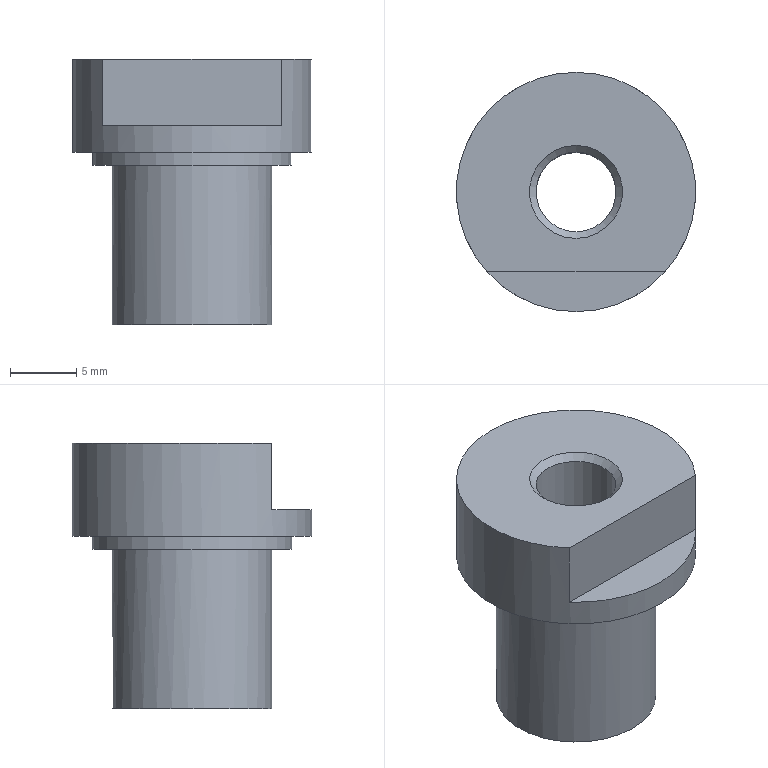Component | NX | REPL_DRILL_BUSH | 1 solid | 12 faces | box 18 x 18 x 20 mm | volume 2605 mm3 | plane 6 | cylinder 4 | cone 2 | commonest cylinder face diameters 12 x1 15 x1 18 x1 6 x1
STEP:
#1=CARTESIAN_POINT('',(0.,0.,0.));
#2=DIRECTION('',(0.,0.,1.));
#3=DIRECTION('',(1.,0.,0.));
#4=AXIS2_PLACEMENT_3D('',#1,#2,#3);
#5=CARTESIAN_POINT('',(11.228,-14.027,-173.719));
#6=VERTEX_POINT('',#5);
#7=CARTESIAN_POINT('',(11.228,-17.527,-173.719));
#8=DIRECTION('',(0.,0.,1.));
#9=DIRECTION('',(0.,1.,0.));
#10=AXIS2_PLACEMENT_3D('',#7,#8,#9);
#11=CIRCLE('',#10,3.5);
#12=CARTESIAN_POINT('',(11.228,-17.527,-173.719));
#13=DIRECTION('',(0.,0.,-1.));
#14=DIRECTION('',(0.,1.,0.));
#15=AXIS2_PLACEMENT_3D('',#12,#13,#14);
#16=PLANE('',#15);
#17=CARTESIAN_POINT('',(3.5,0.));
#18=CARTESIAN_POINT('',(3.5,-6.062));
#19=CARTESIAN_POINT('',(-1.75,-3.031));
#20=CARTESIAN_POINT('',(-7.,-0.));
#21=CARTESIAN_POINT('',(-1.75,3.031));
#22=CARTESIAN_POINT('',(3.5,6.062));
#23=CARTESIAN_POINT('',(3.5,0.));
#24=(BOUNDED_CURVE()B_SPLINE_CURVE(2,(#17,#18,#19,#20,#21,#22,#23),.UNSPECIFIED.,.T.,.F.)B_SPLINE_CURVE_WITH_KNOTS((1,2,2,2,2,1),(-2.094,0.,2.094,4.189,6.283,8.378),.UNSPECIFIED.)CURVE()GEOMETRIC_REPRESENTATION_ITEM()RATIONAL_B_SPLINE_CURVE((1.,0.5,1.,0.5,1.,0.5,1.))REPRESENTATION_ITEM(''));
#25=(GEOMETRIC_REPRESENTATION_CONTEXT(2)PARAMETRIC_REPRESENTATION_CONTEXT()REPRESENTATION_CONTEXT('',''));
#26=DEFINITIONAL_REPRESENTATION('',(#24),#25);
#27=PCURVE('',#16,#26);
#28=CARTESIAN_POINT('',(11.228,-17.527,-173.219));
#29=DIRECTION('',(0.,0.,-1.));
#30=DIRECTION('',(0.,1.,0.));
#31=AXIS2_PLACEMENT_3D('',#28,#29,#30);
#32=CONICAL_SURFACE('',#31,3.,0.7854);
#33=CARTESIAN_POINT('',(6.283,0.5));
#34=DIRECTION('',(-1.,0.));
#35=VECTOR('',#34,1.);
#36=LINE('',#33,#35);
#37=(GEOMETRIC_REPRESENTATION_CONTEXT(2)PARAMETRIC_REPRESENTATION_CONTEXT()REPRESENTATION_CONTEXT('',''));
#38=DEFINITIONAL_REPRESENTATION('',(#36),#37);
#39=PCURVE('',#32,#38);
#40=SURFACE_CURVE('',#11,(#27,#39),.PCURVE_S1.);
#41=EDGE_CURVE('',#6,#6,#40,.T.);
#42=ORIENTED_EDGE('',*,*,#41,.T.);
#43=EDGE_LOOP('',(#42));
#44=FACE_BOUND('',#43,.T.);
#45=CARTESIAN_POINT('',(11.228,-23.527,-173.719));
#46=VERTEX_POINT('',#45);
#47=CARTESIAN_POINT('',(11.228,-17.527,-173.719));
#48=DIRECTION('',(0.,0.,1.));
#49=DIRECTION('',(0.,-1.,0.));
#50=AXIS2_PLACEMENT_3D('',#47,#48,#49);
#51=CIRCLE('',#50,6.);
#52=CARTESIAN_POINT('',(-6.,0.));
#53=CARTESIAN_POINT('',(-6.,10.392));
#54=CARTESIAN_POINT('',(3.,5.196));
#55=CARTESIAN_POINT('',(12.,0.));
#56=CARTESIAN_POINT('',(3.,-5.196));
#57=CARTESIAN_POINT('',(-6.,-10.392));
#58=CARTESIAN_POINT('',(-6.,0.));
#59=(BOUNDED_CURVE()B_SPLINE_CURVE(2,(#52,#53,#54,#55,#56,#57,#58),.UNSPECIFIED.,.T.,.F.)B_SPLINE_CURVE_WITH_KNOTS((1,2,2,2,2,1),(-2.094,0.,2.094,4.189,6.283,8.378),.UNSPECIFIED.)CURVE()GEOMETRIC_REPRESENTATION_ITEM()RATIONAL_B_SPLINE_CURVE((1.,0.5,1.,0.5,1.,0.5,1.))REPRESENTATION_ITEM(''));
#60=(GEOMETRIC_REPRESENTATION_CONTEXT(2)PARAMETRIC_REPRESENTATION_CONTEXT()REPRESENTATION_CONTEXT('',''));
#61=DEFINITIONAL_REPRESENTATION('',(#59),#60);
#62=PCURVE('',#16,#61);
#63=CARTESIAN_POINT('',(11.228,-17.527,-173.719));
#64=DIRECTION('',(0.,0.,1.));
#65=DIRECTION('',(0.,-1.,0.));
#66=AXIS2_PLACEMENT_3D('',#63,#64,#65);
#67=CYLINDRICAL_SURFACE('',#66,6.);
#68=CARTESIAN_POINT('',(0.,0.));
#69=DIRECTION('',(1.,0.));
#70=VECTOR('',#69,1.);
#71=LINE('',#68,#70);
#72=(GEOMETRIC_REPRESENTATION_CONTEXT(2)PARAMETRIC_REPRESENTATION_CONTEXT()REPRESENTATION_CONTEXT('',''));
#73=DEFINITIONAL_REPRESENTATION('',(#71),#72);
#74=PCURVE('',#67,#73);
#75=SURFACE_CURVE('',#51,(#62,#74),.PCURVE_S1.);
#76=EDGE_CURVE('',#46,#46,#75,.T.);
#77=ORIENTED_EDGE('',*,*,#76,.F.);
#78=EDGE_LOOP('',(#77));
#79=FACE_BOUND('',#78,.T.);
#80=ADVANCED_FACE('',(#44,#79),#16,.T.);
#81=CARTESIAN_POINT('',(11.228,-23.527,-161.719));
#82=VERTEX_POINT('',#81);
#83=CARTESIAN_POINT('',(11.228,-11.527,-161.719));
#84=VERTEX_POINT('',#83);
#85=CARTESIAN_POINT('',(11.228,-17.527,-161.719));
#86=DIRECTION('',(0.,0.,1.));
#87=DIRECTION('',(0.,1.,0.));
#88=AXIS2_PLACEMENT_3D('',#85,#86,#87);
#89=CIRCLE('',#88,6.);
#90=CARTESIAN_POINT('',(-3.142,12.));
#91=DIRECTION('',(1.,0.));
#92=VECTOR('',#91,1.);
#93=LINE('',#90,#92);
#94=(GEOMETRIC_REPRESENTATION_CONTEXT(2)PARAMETRIC_REPRESENTATION_CONTEXT()REPRESENTATION_CONTEXT('',''));
#95=DEFINITIONAL_REPRESENTATION('',(#93),#94);
#96=PCURVE('',#67,#95);
#97=CARTESIAN_POINT('',(11.228,-17.527,-161.719));
#98=DIRECTION('',(0.,0.,-1.));
#99=DIRECTION('',(0.,1.,0.));
#100=AXIS2_PLACEMENT_3D('',#97,#98,#99);
#101=PLANE('',#100);
#102=CARTESIAN_POINT('',(6.,0.));
#103=CARTESIAN_POINT('',(6.,-10.392));
#104=CARTESIAN_POINT('',(-3.,-5.196));
#105=CARTESIAN_POINT('',(-12.,-0.));
#106=CARTESIAN_POINT('',(-3.,5.196));
#107=CARTESIAN_POINT('',(6.,10.392));
#108=CARTESIAN_POINT('',(6.,0.));
#109=(BOUNDED_CURVE()B_SPLINE_CURVE(2,(#102,#103,#104,#105,#106,#107,#108),.UNSPECIFIED.,.T.,.F.)B_SPLINE_CURVE_WITH_KNOTS((1,2,2,2,2,1),(-2.094,0.,2.094,4.189,6.283,8.378),.UNSPECIFIED.)CURVE()GEOMETRIC_REPRESENTATION_ITEM()RATIONAL_B_SPLINE_CURVE((1.,0.5,1.,0.5,1.,0.5,1.))REPRESENTATION_ITEM(''));
#110=(GEOMETRIC_REPRESENTATION_CONTEXT(2)PARAMETRIC_REPRESENTATION_CONTEXT()REPRESENTATION_CONTEXT('',''));
#111=DEFINITIONAL_REPRESENTATION('',(#109),#110);
#112=PCURVE('',#101,#111);
#113=SURFACE_CURVE('',#89,(#96,#112),.PCURVE_S1.);
#114=EDGE_CURVE('',#82,#84,#113,.T.);
#115=ORIENTED_EDGE('',*,*,#114,.F.);
#116=CARTESIAN_POINT('',(11.228,-23.527,-173.719));
#117=CARTESIAN_POINT('',(11.228,-23.527,-161.719));
#118=B_SPLINE_CURVE_WITH_KNOTS('',1,(#116,#117),.UNSPECIFIED.,.F.,.F.,(2,2),(0.,12.),.PIECEWISE_BEZIER_KNOTS.);
#119=CARTESIAN_POINT('',(0.,0.));
#120=DIRECTION('',(0.,1.));
#121=VECTOR('',#120,1.);
#122=LINE('',#119,#121);
#123=(GEOMETRIC_REPRESENTATION_CONTEXT(2)PARAMETRIC_REPRESENTATION_CONTEXT()REPRESENTATION_CONTEXT('',''));
#124=DEFINITIONAL_REPRESENTATION('',(#122),#123);
#125=PCURVE('',#67,#124);
#126=CARTESIAN_POINT('',(6.283,0.));
#127=DIRECTION('',(0.,1.));
#128=VECTOR('',#127,1.);
#129=LINE('',#126,#128);
#130=(GEOMETRIC_REPRESENTATION_CONTEXT(2)PARAMETRIC_REPRESENTATION_CONTEXT()REPRESENTATION_CONTEXT('',''));
#131=DEFINITIONAL_REPRESENTATION('',(#129),#130);
#132=PCURVE('',#67,#131);
#133=SEAM_CURVE('',#118,(#125,#132),.PCURVE_S1.);
#134=EDGE_CURVE('',#46,#82,#133,.T.);
#135=ORIENTED_EDGE('',*,*,#134,.F.);
#136=ORIENTED_EDGE('',*,*,#76,.T.);
#137=ORIENTED_EDGE('',*,*,#134,.T.);
#138=CARTESIAN_POINT('',(11.228,-17.527,-161.719));
#139=DIRECTION('',(0.,0.,1.));
#140=DIRECTION('',(0.,1.,0.));
#141=AXIS2_PLACEMENT_3D('',#138,#139,#140);
#142=CIRCLE('',#141,6.);
#143=CARTESIAN_POINT('',(3.142,12.));
#144=DIRECTION('',(1.,0.));
#145=VECTOR('',#144,1.);
#146=LINE('',#143,#145);
#147=(GEOMETRIC_REPRESENTATION_CONTEXT(2)PARAMETRIC_REPRESENTATION_CONTEXT()REPRESENTATION_CONTEXT('',''));
#148=DEFINITIONAL_REPRESENTATION('',(#146),#147);
#149=PCURVE('',#67,#148);
#150=CARTESIAN_POINT('',(6.,0.));
#151=CARTESIAN_POINT('',(6.,-10.392));
#152=CARTESIAN_POINT('',(-3.,-5.196));
#153=CARTESIAN_POINT('',(-12.,-0.));
#154=CARTESIAN_POINT('',(-3.,5.196));
#155=CARTESIAN_POINT('',(6.,10.392));
#156=CARTESIAN_POINT('',(6.,0.));
#157=(BOUNDED_CURVE()B_SPLINE_CURVE(2,(#150,#151,#152,#153,#154,#155,#156),.UNSPECIFIED.,.T.,.F.)B_SPLINE_CURVE_WITH_KNOTS((1,2,2,2,2,1),(-2.094,0.,2.094,4.189,6.283,8.378),.UNSPECIFIED.)CURVE()GEOMETRIC_REPRESENTATION_ITEM()RATIONAL_B_SPLINE_CURVE((1.,0.5,1.,0.5,1.,0.5,1.))REPRESENTATION_ITEM(''));
#158=(GEOMETRIC_REPRESENTATION_CONTEXT(2)PARAMETRIC_REPRESENTATION_CONTEXT()REPRESENTATION_CONTEXT('',''));
#159=DEFINITIONAL_REPRESENTATION('',(#157),#158);
#160=PCURVE('',#101,#159);
#161=SURFACE_CURVE('',#142,(#149,#160),.PCURVE_S1.);
#162=EDGE_CURVE('',#84,#82,#161,.T.);
#163=ORIENTED_EDGE('',*,*,#162,.F.);
#164=EDGE_LOOP('',(#115,#135,#136,#137,#163));
#165=FACE_BOUND('',#164,.T.);
#166=ADVANCED_FACE('',(#165),#67,.T.);
#167=ORIENTED_EDGE('',*,*,#162,.T.);
#168=ORIENTED_EDGE('',*,*,#114,.T.);
#169=EDGE_LOOP('',(#167,#168));
#170=FACE_BOUND('',#169,.T.);
#171=CARTESIAN_POINT('',(11.228,-25.027,-161.719));
#172=VERTEX_POINT('',#171);
#173=CARTESIAN_POINT('',(11.228,-17.527,-161.719));
#174=DIRECTION('',(0.,0.,1.));
#175=DIRECTION('',(0.,-1.,0.));
#176=AXIS2_PLACEMENT_3D('',#173,#174,#175);
#177=CIRCLE('',#176,7.5);
#178=CARTESIAN_POINT('',(-7.5,0.));
#179=CARTESIAN_POINT('',(-7.5,12.99));
#180=CARTESIAN_POINT('',(3.75,6.495));
#181=CARTESIAN_POINT('',(15.,0.));
#182=CARTESIAN_POINT('',(3.75,-6.495));
#183=CARTESIAN_POINT('',(-7.5,-12.99));
#184=CARTESIAN_POINT('',(-7.5,0.));
#185=(BOUNDED_CURVE()B_SPLINE_CURVE(2,(#178,#179,#180,#181,#182,#183,#184),.UNSPECIFIED.,.T.,.F.)B_SPLINE_CURVE_WITH_KNOTS((1,2,2,2,2,1),(-2.094,0.,2.094,4.189,6.283,8.378),.UNSPECIFIED.)CURVE()GEOMETRIC_REPRESENTATION_ITEM()RATIONAL_B_SPLINE_CURVE((1.,0.5,1.,0.5,1.,0.5,1.))REPRESENTATION_ITEM(''));
#186=(GEOMETRIC_REPRESENTATION_CONTEXT(2)PARAMETRIC_REPRESENTATION_CONTEXT()REPRESENTATION_CONTEXT('',''));
#187=DEFINITIONAL_REPRESENTATION('',(#185),#186);
#188=PCURVE('',#101,#187);
#189=CARTESIAN_POINT('',(11.228,-17.527,-161.719));
#190=DIRECTION('',(0.,0.,1.));
#191=DIRECTION('',(0.,-1.,0.));
#192=AXIS2_PLACEMENT_3D('',#189,#190,#191);
#193=CYLINDRICAL_SURFACE('',#192,7.5);
#194=CARTESIAN_POINT('',(0.,0.));
#195=DIRECTION('',(1.,0.));
#196=VECTOR('',#195,1.);
#197=LINE('',#194,#196);
#198=(GEOMETRIC_REPRESENTATION_CONTEXT(2)PARAMETRIC_REPRESENTATION_CONTEXT()REPRESENTATION_CONTEXT('',''));
#199=DEFINITIONAL_REPRESENTATION('',(#197),#198);
#200=PCURVE('',#193,#199);
#201=SURFACE_CURVE('',#177,(#188,#200),.PCURVE_S1.);
#202=EDGE_CURVE('',#172,#172,#201,.T.);
#203=ORIENTED_EDGE('',*,*,#202,.F.);
#204=EDGE_LOOP('',(#203));
#205=FACE_BOUND('',#204,.T.);
#206=ADVANCED_FACE('',(#170,#205),#101,.T.);
#207=CARTESIAN_POINT('',(11.228,-25.027,-160.719));
#208=VERTEX_POINT('',#207);
#209=CARTESIAN_POINT('',(11.228,-10.027,-160.719));
#210=VERTEX_POINT('',#209);
#211=CARTESIAN_POINT('',(11.228,-17.527,-160.719));
#212=DIRECTION('',(0.,0.,1.));
#213=DIRECTION('',(0.,1.,0.));
#214=AXIS2_PLACEMENT_3D('',#211,#212,#213);
#215=CIRCLE('',#214,7.5);
#216=CARTESIAN_POINT('',(-3.142,1.));
#217=DIRECTION('',(1.,0.));
#218=VECTOR('',#217,1.);
#219=LINE('',#216,#218);
#220=(GEOMETRIC_REPRESENTATION_CONTEXT(2)PARAMETRIC_REPRESENTATION_CONTEXT()REPRESENTATION_CONTEXT('',''));
#221=DEFINITIONAL_REPRESENTATION('',(#219),#220);
#222=PCURVE('',#193,#221);
#223=CARTESIAN_POINT('',(11.228,-17.527,-160.719));
#224=DIRECTION('',(0.,0.,-1.));
#225=DIRECTION('',(0.,1.,0.));
#226=AXIS2_PLACEMENT_3D('',#223,#224,#225);
#227=PLANE('',#226);
#228=CARTESIAN_POINT('',(7.5,0.));
#229=CARTESIAN_POINT('',(7.5,-12.99));
#230=CARTESIAN_POINT('',(-3.75,-6.495));
#231=CARTESIAN_POINT('',(-15.,-0.));
#232=CARTESIAN_POINT('',(-3.75,6.495));
#233=CARTESIAN_POINT('',(7.5,12.99));
#234=CARTESIAN_POINT('',(7.5,0.));
#235=(BOUNDED_CURVE()B_SPLINE_CURVE(2,(#228,#229,#230,#231,#232,#233,#234),.UNSPECIFIED.,.T.,.F.)B_SPLINE_CURVE_WITH_KNOTS((1,2,2,2,2,1),(-2.094,0.,2.094,4.189,6.283,8.378),.UNSPECIFIED.)CURVE()GEOMETRIC_REPRESENTATION_ITEM()RATIONAL_B_SPLINE_CURVE((1.,0.5,1.,0.5,1.,0.5,1.))REPRESENTATION_ITEM(''));
#236=(GEOMETRIC_REPRESENTATION_CONTEXT(2)PARAMETRIC_REPRESENTATION_CONTEXT()REPRESENTATION_CONTEXT('',''));
#237=DEFINITIONAL_REPRESENTATION('',(#235),#236);
#238=PCURVE('',#227,#237);
#239=SURFACE_CURVE('',#215,(#222,#238),.PCURVE_S1.);
#240=EDGE_CURVE('',#208,#210,#239,.T.);
#241=ORIENTED_EDGE('',*,*,#240,.F.);
#242=CARTESIAN_POINT('',(11.228,-25.027,-161.719));
#243=CARTESIAN_POINT('',(11.228,-25.027,-160.719));
#244=B_SPLINE_CURVE_WITH_KNOTS('',1,(#242,#243),.UNSPECIFIED.,.F.,.F.,(2,2),(0.,1.),.PIECEWISE_BEZIER_KNOTS.);
#245=CARTESIAN_POINT('',(0.,0.));
#246=DIRECTION('',(0.,1.));
#247=VECTOR('',#246,1.);
#248=LINE('',#245,#247);
#249=(GEOMETRIC_REPRESENTATION_CONTEXT(2)PARAMETRIC_REPRESENTATION_CONTEXT()REPRESENTATION_CONTEXT('',''));
#250=DEFINITIONAL_REPRESENTATION('',(#248),#249);
#251=PCURVE('',#193,#250);
#252=CARTESIAN_POINT('',(6.283,0.));
#253=DIRECTION('',(0.,1.));
#254=VECTOR('',#253,1.);
#255=LINE('',#252,#254);
#256=(GEOMETRIC_REPRESENTATION_CONTEXT(2)PARAMETRIC_REPRESENTATION_CONTEXT()REPRESENTATION_CONTEXT('',''));
#257=DEFINITIONAL_REPRESENTATION('',(#255),#256);
#258=PCURVE('',#193,#257);
#259=SEAM_CURVE('',#244,(#251,#258),.PCURVE_S1.);
#260=EDGE_CURVE('',#172,#208,#259,.T.);
#261=ORIENTED_EDGE('',*,*,#260,.F.);
#262=ORIENTED_EDGE('',*,*,#202,.T.);
#263=ORIENTED_EDGE('',*,*,#260,.T.);
#264=CARTESIAN_POINT('',(11.228,-17.527,-160.719));
#265=DIRECTION('',(0.,0.,1.));
#266=DIRECTION('',(0.,1.,0.));
#267=AXIS2_PLACEMENT_3D('',#264,#265,#266);
#268=CIRCLE('',#267,7.5);
#269=CARTESIAN_POINT('',(3.142,1.));
#270=DIRECTION('',(1.,0.));
#271=VECTOR('',#270,1.);
#272=LINE('',#269,#271);
#273=(GEOMETRIC_REPRESENTATION_CONTEXT(2)PARAMETRIC_REPRESENTATION_CONTEXT()REPRESENTATION_CONTEXT('',''));
#274=DEFINITIONAL_REPRESENTATION('',(#272),#273);
#275=PCURVE('',#193,#274);
#276=CARTESIAN_POINT('',(7.5,0.));
#277=CARTESIAN_POINT('',(7.5,-12.99));
#278=CARTESIAN_POINT('',(-3.75,-6.495));
#279=CARTESIAN_POINT('',(-15.,-0.));
#280=CARTESIAN_POINT('',(-3.75,6.495));
#281=CARTESIAN_POINT('',(7.5,12.99));
#282=CARTESIAN_POINT('',(7.5,0.));
#283=(BOUNDED_CURVE()B_SPLINE_CURVE(2,(#276,#277,#278,#279,#280,#281,#282),.UNSPECIFIED.,.T.,.F.)B_SPLINE_CURVE_WITH_KNOTS((1,2,2,2,2,1),(-2.094,0.,2.094,4.189,6.283,8.378),.UNSPECIFIED.)CURVE()GEOMETRIC_REPRESENTATION_ITEM()RATIONAL_B_SPLINE_CURVE((1.,0.5,1.,0.5,1.,0.5,1.))REPRESENTATION_ITEM(''));
#284=(GEOMETRIC_REPRESENTATION_CONTEXT(2)PARAMETRIC_REPRESENTATION_CONTEXT()REPRESENTATION_CONTEXT('',''));
#285=DEFINITIONAL_REPRESENTATION('',(#283),#284);
#286=PCURVE('',#227,#285);
#287=SURFACE_CURVE('',#268,(#275,#286),.PCURVE_S1.);
#288=EDGE_CURVE('',#210,#208,#287,.T.);
#289=ORIENTED_EDGE('',*,*,#288,.F.);
#290=EDGE_LOOP('',(#241,#261,#262,#263,#289));
#291=FACE_BOUND('',#290,.T.);
#292=ADVANCED_FACE('',(#291),#193,.T.);
#293=CARTESIAN_POINT('',(11.228,-21.027,-153.719));
#294=VERTEX_POINT('',#293);
#295=CARTESIAN_POINT('',(11.228,-17.527,-153.719));
#296=DIRECTION('',(0.,0.,-1.));
#297=DIRECTION('',(0.,-1.,0.));
#298=AXIS2_PLACEMENT_3D('',#295,#296,#297);
#299=CIRCLE('',#298,3.5);
#300=CARTESIAN_POINT('',(11.228,-17.527,-153.719));
#301=DIRECTION('',(0.,0.,1.));
#302=DIRECTION('',(0.,-1.,0.));
#303=AXIS2_PLACEMENT_3D('',#300,#301,#302);
#304=PLANE('',#303);
#305=CARTESIAN_POINT('',(3.5,0.));
#306=CARTESIAN_POINT('',(3.5,-6.062));
#307=CARTESIAN_POINT('',(-1.75,-3.031));
#308=CARTESIAN_POINT('',(-7.,-0.));
#309=CARTESIAN_POINT('',(-1.75,3.031));
#310=CARTESIAN_POINT('',(3.5,6.062));
#311=CARTESIAN_POINT('',(3.5,0.));
#312=(BOUNDED_CURVE()B_SPLINE_CURVE(2,(#305,#306,#307,#308,#309,#310,#311),.UNSPECIFIED.,.T.,.F.)B_SPLINE_CURVE_WITH_KNOTS((1,2,2,2,2,1),(-2.094,0.,2.094,4.189,6.283,8.378),.UNSPECIFIED.)CURVE()GEOMETRIC_REPRESENTATION_ITEM()RATIONAL_B_SPLINE_CURVE((1.,0.5,1.,0.5,1.,0.5,1.))REPRESENTATION_ITEM(''));
#313=(GEOMETRIC_REPRESENTATION_CONTEXT(2)PARAMETRIC_REPRESENTATION_CONTEXT()REPRESENTATION_CONTEXT('',''));
#314=DEFINITIONAL_REPRESENTATION('',(#312),#313);
#315=PCURVE('',#304,#314);
#316=CARTESIAN_POINT('',(11.228,-17.527,-153.719));
#317=DIRECTION('',(0.,0.,1.));
#318=DIRECTION('',(0.,-1.,0.));
#319=AXIS2_PLACEMENT_3D('',#316,#317,#318);
#320=CONICAL_SURFACE('',#319,3.5,0.7854);
#321=CARTESIAN_POINT('',(6.283,0.));
#322=DIRECTION('',(-1.,0.));
#323=VECTOR('',#322,1.);
#324=LINE('',#321,#323);
#325=(GEOMETRIC_REPRESENTATION_CONTEXT(2)PARAMETRIC_REPRESENTATION_CONTEXT()REPRESENTATION_CONTEXT('',''));
#326=DEFINITIONAL_REPRESENTATION('',(#324),#325);
#327=PCURVE('',#320,#326);
#328=SURFACE_CURVE('',#299,(#315,#327),.PCURVE_S1.);
#329=EDGE_CURVE('',#294,#294,#328,.T.);
#330=ORIENTED_EDGE('',*,*,#329,.T.);
#331=EDGE_LOOP('',(#330));
#332=FACE_BOUND('',#331,.T.);
#333=CARTESIAN_POINT('',(17.936,-23.527,-153.719));
#334=VERTEX_POINT('',#333);
#335=CARTESIAN_POINT('',(4.52,-23.527,-153.719));
#336=VERTEX_POINT('',#335);
#337=CARTESIAN_POINT('',(20.728,-23.527,-153.719));
#338=DIRECTION('',(-1.,0.,0.));
#339=VECTOR('',#338,1.);
#340=LINE('',#337,#339);
#341=CARTESIAN_POINT('',(6.,9.5));
#342=DIRECTION('',(0.,-1.));
#343=VECTOR('',#342,1.);
#344=LINE('',#341,#343);
#345=(GEOMETRIC_REPRESENTATION_CONTEXT(2)PARAMETRIC_REPRESENTATION_CONTEXT()REPRESENTATION_CONTEXT('',''));
#346=DEFINITIONAL_REPRESENTATION('',(#344),#345);
#347=PCURVE('',#304,#346);
#348=CARTESIAN_POINT('',(20.728,-23.527,-158.719));
#349=DIRECTION('',(0.,1.,0.));
#350=DIRECTION('',(0.,0.,1.));
#351=AXIS2_PLACEMENT_3D('',#348,#349,#350);
#352=PLANE('',#351);
#353=CARTESIAN_POINT('',(5.,0.));
#354=DIRECTION('',(0.,-1.));
#355=VECTOR('',#354,1.);
#356=LINE('',#353,#355);
#357=(GEOMETRIC_REPRESENTATION_CONTEXT(2)PARAMETRIC_REPRESENTATION_CONTEXT()REPRESENTATION_CONTEXT('',''));
#358=DEFINITIONAL_REPRESENTATION('',(#356),#357);
#359=PCURVE('',#352,#358);
#360=SURFACE_CURVE('',#340,(#347,#359),.PCURVE_S1.);
#361=EDGE_CURVE('',#334,#336,#360,.T.);
#362=ORIENTED_EDGE('',*,*,#361,.F.);
#363=CARTESIAN_POINT('',(11.228,-17.527,-153.719));
#364=DIRECTION('',(0.,0.,-1.));
#365=DIRECTION('',(0.,-1.,0.));
#366=AXIS2_PLACEMENT_3D('',#363,#364,#365);
#367=CIRCLE('',#366,9.);
#368=CARTESIAN_POINT('',(9.,0.));
#369=CARTESIAN_POINT('',(9.,-15.588));
#370=CARTESIAN_POINT('',(-4.5,-7.794));
#371=CARTESIAN_POINT('',(-18.,-0.));
#372=CARTESIAN_POINT('',(-4.5,7.794));
#373=CARTESIAN_POINT('',(9.,15.588));
#374=CARTESIAN_POINT('',(9.,0.));
#375=(BOUNDED_CURVE()B_SPLINE_CURVE(2,(#368,#369,#370,#371,#372,#373,#374),.UNSPECIFIED.,.T.,.F.)B_SPLINE_CURVE_WITH_KNOTS((1,2,2,2,2,1),(-2.094,0.,2.094,4.189,6.283,8.378),.UNSPECIFIED.)CURVE()GEOMETRIC_REPRESENTATION_ITEM()RATIONAL_B_SPLINE_CURVE((1.,0.5,1.,0.5,1.,0.5,1.))REPRESENTATION_ITEM(''));
#376=(GEOMETRIC_REPRESENTATION_CONTEXT(2)PARAMETRIC_REPRESENTATION_CONTEXT()REPRESENTATION_CONTEXT('',''));
#377=DEFINITIONAL_REPRESENTATION('',(#375),#376);
#378=PCURVE('',#304,#377);
#379=CARTESIAN_POINT('',(11.228,-17.527,-160.719));
#380=DIRECTION('',(0.,0.,1.));
#381=DIRECTION('',(0.,-1.,0.));
#382=AXIS2_PLACEMENT_3D('',#379,#380,#381);
#383=CYLINDRICAL_SURFACE('',#382,9.);
#384=CARTESIAN_POINT('',(6.283,7.));
#385=DIRECTION('',(-1.,0.));
#386=VECTOR('',#385,1.);
#387=LINE('',#384,#386);
#388=(GEOMETRIC_REPRESENTATION_CONTEXT(2)PARAMETRIC_REPRESENTATION_CONTEXT()REPRESENTATION_CONTEXT('',''));
#389=DEFINITIONAL_REPRESENTATION('',(#387),#388);
#390=PCURVE('',#383,#389);
#391=SURFACE_CURVE('',#367,(#378,#390),.PCURVE_S1.);
#392=EDGE_CURVE('',#336,#334,#391,.T.);
#393=ORIENTED_EDGE('',*,*,#392,.F.);
#394=EDGE_LOOP('',(#362,#393));
#395=FACE_BOUND('',#394,.T.);
#396=ADVANCED_FACE('',(#332,#395),#304,.T.);
#397=ORIENTED_EDGE('',*,*,#288,.T.);
#398=ORIENTED_EDGE('',*,*,#240,.T.);
#399=EDGE_LOOP('',(#397,#398));
#400=FACE_BOUND('',#399,.T.);
#401=CARTESIAN_POINT('',(11.228,-26.527,-160.719));
#402=VERTEX_POINT('',#401);
#403=CARTESIAN_POINT('',(11.228,-17.527,-160.719));
#404=DIRECTION('',(0.,0.,1.));
#405=DIRECTION('',(0.,-1.,0.));
#406=AXIS2_PLACEMENT_3D('',#403,#404,#405);
#407=CIRCLE('',#406,9.);
#408=CARTESIAN_POINT('',(-9.,0.));
#409=CARTESIAN_POINT('',(-9.,15.588));
#410=CARTESIAN_POINT('',(4.5,7.794));
#411=CARTESIAN_POINT('',(18.,0.));
#412=CARTESIAN_POINT('',(4.5,-7.794));
#413=CARTESIAN_POINT('',(-9.,-15.588));
#414=CARTESIAN_POINT('',(-9.,0.));
#415=(BOUNDED_CURVE()B_SPLINE_CURVE(2,(#408,#409,#410,#411,#412,#413,#414),.UNSPECIFIED.,.T.,.F.)B_SPLINE_CURVE_WITH_KNOTS((1,2,2,2,2,1),(-2.094,0.,2.094,4.189,6.283,8.378),.UNSPECIFIED.)CURVE()GEOMETRIC_REPRESENTATION_ITEM()RATIONAL_B_SPLINE_CURVE((1.,0.5,1.,0.5,1.,0.5,1.))REPRESENTATION_ITEM(''));
#416=(GEOMETRIC_REPRESENTATION_CONTEXT(2)PARAMETRIC_REPRESENTATION_CONTEXT()REPRESENTATION_CONTEXT('',''));
#417=DEFINITIONAL_REPRESENTATION('',(#415),#416);
#418=PCURVE('',#227,#417);
#419=CARTESIAN_POINT('',(0.,0.));
#420=DIRECTION('',(1.,0.));
#421=VECTOR('',#420,1.);
#422=LINE('',#419,#421);
#423=(GEOMETRIC_REPRESENTATION_CONTEXT(2)PARAMETRIC_REPRESENTATION_CONTEXT()REPRESENTATION_CONTEXT('',''));
#424=DEFINITIONAL_REPRESENTATION('',(#422),#423);
#425=PCURVE('',#383,#424);
#426=SURFACE_CURVE('',#407,(#418,#425),.PCURVE_S1.);
#427=EDGE_CURVE('',#402,#402,#426,.T.);
#428=ORIENTED_EDGE('',*,*,#427,.F.);
#429=EDGE_LOOP('',(#428));
#430=FACE_BOUND('',#429,.T.);
#431=ADVANCED_FACE('',(#400,#430),#227,.T.);
#432=CARTESIAN_POINT('',(4.52,-23.527,-158.719));
#433=VERTEX_POINT('',#432);
#434=CARTESIAN_POINT('',(4.52,-23.527,-160.719));
#435=DIRECTION('',(0.,0.,-1.));
#436=VECTOR('',#435,1.);
#437=LINE('',#434,#436);
#438=CARTESIAN_POINT('',(5.442,0.));
#439=DIRECTION('',(0.,-1.));
#440=VECTOR('',#439,1.);
#441=LINE('',#438,#440);
#442=(GEOMETRIC_REPRESENTATION_CONTEXT(2)PARAMETRIC_REPRESENTATION_CONTEXT()REPRESENTATION_CONTEXT('',''));
#443=DEFINITIONAL_REPRESENTATION('',(#441),#442);
#444=PCURVE('',#383,#443);
#445=CARTESIAN_POINT('',(-2.,-16.208));
#446=DIRECTION('',(-1.,0.));
#447=VECTOR('',#446,1.);
#448=LINE('',#445,#447);
#449=(GEOMETRIC_REPRESENTATION_CONTEXT(2)PARAMETRIC_REPRESENTATION_CONTEXT()REPRESENTATION_CONTEXT('',''));
#450=DEFINITIONAL_REPRESENTATION('',(#448),#449);
#451=PCURVE('',#352,#450);
#452=SURFACE_CURVE('',#437,(#444,#451),.PCURVE_S1.);
#453=EDGE_CURVE('',#336,#433,#452,.T.);
#454=ORIENTED_EDGE('',*,*,#453,.F.);
#455=ORIENTED_EDGE('',*,*,#392,.T.);
#456=CARTESIAN_POINT('',(17.936,-23.527,-158.719));
#457=VERTEX_POINT('',#456);
#458=CARTESIAN_POINT('',(17.936,-23.527,-160.719));
#459=DIRECTION('',(0.,0.,1.));
#460=VECTOR('',#459,1.);
#461=LINE('',#458,#460);
#462=CARTESIAN_POINT('',(0.8411,0.));
#463=DIRECTION('',(0.,1.));
#464=VECTOR('',#463,1.);
#465=LINE('',#462,#464);
#466=(GEOMETRIC_REPRESENTATION_CONTEXT(2)PARAMETRIC_REPRESENTATION_CONTEXT()REPRESENTATION_CONTEXT('',''));
#467=DEFINITIONAL_REPRESENTATION('',(#465),#466);
#468=PCURVE('',#383,#467);
#469=CARTESIAN_POINT('',(-2.,-2.792));
#470=DIRECTION('',(1.,0.));
#471=VECTOR('',#470,1.);
#472=LINE('',#469,#471);
#473=(GEOMETRIC_REPRESENTATION_CONTEXT(2)PARAMETRIC_REPRESENTATION_CONTEXT()REPRESENTATION_CONTEXT('',''));
#474=DEFINITIONAL_REPRESENTATION('',(#472),#473);
#475=PCURVE('',#352,#474);
#476=SURFACE_CURVE('',#461,(#468,#475),.PCURVE_S1.);
#477=EDGE_CURVE('',#457,#334,#476,.T.);
#478=ORIENTED_EDGE('',*,*,#477,.F.);
#479=CARTESIAN_POINT('',(11.228,-26.527,-158.719));
#480=VERTEX_POINT('',#479);
#481=CARTESIAN_POINT('',(11.228,-17.527,-158.719));
#482=DIRECTION('',(0.,0.,-1.));
#483=DIRECTION('',(0.,-1.,0.));
#484=AXIS2_PLACEMENT_3D('',#481,#482,#483);
#485=CIRCLE('',#484,9.);
#486=CARTESIAN_POINT('',(6.283,2.));
#487=DIRECTION('',(-1.,0.));
#488=VECTOR('',#487,1.);
#489=LINE('',#486,#488);
#490=(GEOMETRIC_REPRESENTATION_CONTEXT(2)PARAMETRIC_REPRESENTATION_CONTEXT()REPRESENTATION_CONTEXT('',''));
#491=DEFINITIONAL_REPRESENTATION('',(#489),#490);
#492=PCURVE('',#383,#491);
#493=CARTESIAN_POINT('',(11.228,-17.527,-158.719));
#494=DIRECTION('',(0.,0.,1.));
#495=DIRECTION('',(0.,-1.,0.));
#496=AXIS2_PLACEMENT_3D('',#493,#494,#495);
#497=PLANE('',#496);
#498=CARTESIAN_POINT('',(9.,0.));
#499=CARTESIAN_POINT('',(9.,-15.588));
#500=CARTESIAN_POINT('',(-4.5,-7.794));
#501=CARTESIAN_POINT('',(-18.,-0.));
#502=CARTESIAN_POINT('',(-4.5,7.794));
#503=CARTESIAN_POINT('',(9.,15.588));
#504=CARTESIAN_POINT('',(9.,0.));
#505=(BOUNDED_CURVE()B_SPLINE_CURVE(2,(#498,#499,#500,#501,#502,#503,#504),.UNSPECIFIED.,.T.,.F.)B_SPLINE_CURVE_WITH_KNOTS((1,2,2,2,2,1),(-2.094,0.,2.094,4.189,6.283,8.378),.UNSPECIFIED.)CURVE()GEOMETRIC_REPRESENTATION_ITEM()RATIONAL_B_SPLINE_CURVE((1.,0.5,1.,0.5,1.,0.5,1.))REPRESENTATION_ITEM(''));
#506=(GEOMETRIC_REPRESENTATION_CONTEXT(2)PARAMETRIC_REPRESENTATION_CONTEXT()REPRESENTATION_CONTEXT('',''));
#507=DEFINITIONAL_REPRESENTATION('',(#505),#506);
#508=PCURVE('',#497,#507);
#509=SURFACE_CURVE('',#485,(#492,#508),.PCURVE_S1.);
#510=EDGE_CURVE('',#457,#480,#509,.T.);
#511=ORIENTED_EDGE('',*,*,#510,.T.);
#512=CARTESIAN_POINT('',(11.228,-26.527,-160.719));
#513=CARTESIAN_POINT('',(11.228,-26.527,-158.719));
#514=B_SPLINE_CURVE_WITH_KNOTS('',1,(#512,#513),.UNSPECIFIED.,.F.,.F.,(2,2),(0.,2.),.PIECEWISE_BEZIER_KNOTS.);
#515=CARTESIAN_POINT('',(0.,0.));
#516=DIRECTION('',(0.,1.));
#517=VECTOR('',#516,1.);
#518=LINE('',#515,#517);
#519=(GEOMETRIC_REPRESENTATION_CONTEXT(2)PARAMETRIC_REPRESENTATION_CONTEXT()REPRESENTATION_CONTEXT('',''));
#520=DEFINITIONAL_REPRESENTATION('',(#518),#519);
#521=PCURVE('',#383,#520);
#522=CARTESIAN_POINT('',(6.283,0.));
#523=DIRECTION('',(0.,1.));
#524=VECTOR('',#523,1.);
#525=LINE('',#522,#524);
#526=(GEOMETRIC_REPRESENTATION_CONTEXT(2)PARAMETRIC_REPRESENTATION_CONTEXT()REPRESENTATION_CONTEXT('',''));
#527=DEFINITIONAL_REPRESENTATION('',(#525),#526);
#528=PCURVE('',#383,#527);
#529=SEAM_CURVE('',#514,(#521,#528),.PCURVE_S1.);
#530=EDGE_CURVE('',#402,#480,#529,.T.);
#531=ORIENTED_EDGE('',*,*,#530,.F.);
#532=ORIENTED_EDGE('',*,*,#427,.T.);
#533=ORIENTED_EDGE('',*,*,#530,.T.);
#534=CARTESIAN_POINT('',(11.228,-17.527,-158.719));
#535=DIRECTION('',(0.,0.,-1.));
#536=DIRECTION('',(0.,-1.,0.));
#537=AXIS2_PLACEMENT_3D('',#534,#535,#536);
#538=CIRCLE('',#537,9.);
#539=CARTESIAN_POINT('',(12.566,2.));
#540=DIRECTION('',(-1.,0.));
#541=VECTOR('',#540,1.);
#542=LINE('',#539,#541);
#543=(GEOMETRIC_REPRESENTATION_CONTEXT(2)PARAMETRIC_REPRESENTATION_CONTEXT()REPRESENTATION_CONTEXT('',''));
#544=DEFINITIONAL_REPRESENTATION('',(#542),#543);
#545=PCURVE('',#383,#544);
#546=CARTESIAN_POINT('',(9.,0.));
#547=CARTESIAN_POINT('',(9.,-15.588));
#548=CARTESIAN_POINT('',(-4.5,-7.794));
#549=CARTESIAN_POINT('',(-18.,-0.));
#550=CARTESIAN_POINT('',(-4.5,7.794));
#551=CARTESIAN_POINT('',(9.,15.588));
#552=CARTESIAN_POINT('',(9.,0.));
#553=(BOUNDED_CURVE()B_SPLINE_CURVE(2,(#546,#547,#548,#549,#550,#551,#552),.UNSPECIFIED.,.T.,.F.)B_SPLINE_CURVE_WITH_KNOTS((1,2,2,2,2,1),(-2.094,0.,2.094,4.189,6.283,8.378),.UNSPECIFIED.)CURVE()GEOMETRIC_REPRESENTATION_ITEM()RATIONAL_B_SPLINE_CURVE((1.,0.5,1.,0.5,1.,0.5,1.))REPRESENTATION_ITEM(''));
#554=(GEOMETRIC_REPRESENTATION_CONTEXT(2)PARAMETRIC_REPRESENTATION_CONTEXT()REPRESENTATION_CONTEXT('',''));
#555=DEFINITIONAL_REPRESENTATION('',(#553),#554);
#556=PCURVE('',#497,#555);
#557=SURFACE_CURVE('',#538,(#545,#556),.PCURVE_S1.);
#558=EDGE_CURVE('',#480,#433,#557,.T.);
#559=ORIENTED_EDGE('',*,*,#558,.T.);
#560=EDGE_LOOP('',(#454,#455,#478,#511,#531,#532,#533,#559));
#561=FACE_BOUND('',#560,.T.);
#562=ADVANCED_FACE('',(#561),#383,.T.);
#563=CARTESIAN_POINT('',(11.228,-14.527,-173.219));
#564=VERTEX_POINT('',#563);
#565=CARTESIAN_POINT('',(11.228,-17.527,-173.219));
#566=DIRECTION('',(0.,0.,-1.));
#567=DIRECTION('',(0.,1.,0.));
#568=AXIS2_PLACEMENT_3D('',#565,#566,#567);
#569=CIRCLE('',#568,3.);
#570=CARTESIAN_POINT('',(11.228,-17.527,-153.719));
#571=DIRECTION('',(0.,0.,-1.));
#572=DIRECTION('',(0.,1.,0.));
#573=AXIS2_PLACEMENT_3D('',#570,#571,#572);
#574=CYLINDRICAL_SURFACE('',#573,3.);
#575=CARTESIAN_POINT('',(0.,19.5));
#576=DIRECTION('',(1.,0.));
#577=VECTOR('',#576,1.);
#578=LINE('',#575,#577);
#579=(GEOMETRIC_REPRESENTATION_CONTEXT(2)PARAMETRIC_REPRESENTATION_CONTEXT()REPRESENTATION_CONTEXT('',''));
#580=DEFINITIONAL_REPRESENTATION('',(#578),#579);
#581=PCURVE('',#574,#580);
#582=CARTESIAN_POINT('',(0.,0.));
#583=DIRECTION('',(1.,0.));
#584=VECTOR('',#583,1.);
#585=LINE('',#582,#584);
#586=(GEOMETRIC_REPRESENTATION_CONTEXT(2)PARAMETRIC_REPRESENTATION_CONTEXT()REPRESENTATION_CONTEXT('',''));
#587=DEFINITIONAL_REPRESENTATION('',(#585),#586);
#588=PCURVE('',#32,#587);
#589=SURFACE_CURVE('',#569,(#581,#588),.PCURVE_S1.);
#590=EDGE_CURVE('',#564,#564,#589,.T.);
#591=ORIENTED_EDGE('',*,*,#590,.F.);
#592=CARTESIAN_POINT('',(11.228,-14.527,-154.219));
#593=VERTEX_POINT('',#592);
#594=CARTESIAN_POINT('',(11.228,-14.527,-154.219));
#595=CARTESIAN_POINT('',(11.228,-14.527,-173.219));
#596=B_SPLINE_CURVE_WITH_KNOTS('',1,(#594,#595),.UNSPECIFIED.,.F.,.F.,(2,2),(0.5,19.5),.PIECEWISE_BEZIER_KNOTS.);
#597=CARTESIAN_POINT('',(0.,0.));
#598=DIRECTION('',(0.,1.));
#599=VECTOR('',#598,1.);
#600=LINE('',#597,#599);
#601=(GEOMETRIC_REPRESENTATION_CONTEXT(2)PARAMETRIC_REPRESENTATION_CONTEXT()REPRESENTATION_CONTEXT('',''));
#602=DEFINITIONAL_REPRESENTATION('',(#600),#601);
#603=PCURVE('',#574,#602);
#604=CARTESIAN_POINT('',(6.283,0.));
#605=DIRECTION('',(0.,1.));
#606=VECTOR('',#605,1.);
#607=LINE('',#604,#606);
#608=(GEOMETRIC_REPRESENTATION_CONTEXT(2)PARAMETRIC_REPRESENTATION_CONTEXT()REPRESENTATION_CONTEXT('',''));
#609=DEFINITIONAL_REPRESENTATION('',(#607),#608);
#610=PCURVE('',#574,#609);
#611=SEAM_CURVE('',#596,(#603,#610),.PCURVE_S1.);
#612=EDGE_CURVE('',#593,#564,#611,.T.);
#613=ORIENTED_EDGE('',*,*,#612,.F.);
#614=CARTESIAN_POINT('',(11.228,-20.527,-154.219));
#615=VERTEX_POINT('',#614);
#616=CARTESIAN_POINT('',(11.228,-17.527,-154.219));
#617=DIRECTION('',(0.,0.,1.));
#618=DIRECTION('',(0.,-1.,0.));
#619=AXIS2_PLACEMENT_3D('',#616,#617,#618);
#620=CIRCLE('',#619,3.);
#621=CARTESIAN_POINT('',(3.142,0.5));
#622=DIRECTION('',(-1.,0.));
#623=VECTOR('',#622,1.);
#624=LINE('',#621,#623);
#625=(GEOMETRIC_REPRESENTATION_CONTEXT(2)PARAMETRIC_REPRESENTATION_CONTEXT()REPRESENTATION_CONTEXT('',''));
#626=DEFINITIONAL_REPRESENTATION('',(#624),#625);
#627=PCURVE('',#574,#626);
#628=CARTESIAN_POINT('',(0.,-0.5));
#629=DIRECTION('',(1.,0.));
#630=VECTOR('',#629,1.);
#631=LINE('',#628,#630);
#632=(GEOMETRIC_REPRESENTATION_CONTEXT(2)PARAMETRIC_REPRESENTATION_CONTEXT()REPRESENTATION_CONTEXT('',''));
#633=DEFINITIONAL_REPRESENTATION('',(#631),#632);
#634=PCURVE('',#320,#633);
#635=SURFACE_CURVE('',#620,(#627,#634),.PCURVE_S1.);
#636=EDGE_CURVE('',#615,#593,#635,.T.);
#637=ORIENTED_EDGE('',*,*,#636,.F.);
#638=CARTESIAN_POINT('',(11.228,-17.527,-154.219));
#639=DIRECTION('',(0.,0.,1.));
#640=DIRECTION('',(0.,-1.,0.));
#641=AXIS2_PLACEMENT_3D('',#638,#639,#640);
#642=CIRCLE('',#641,3.);
#643=CARTESIAN_POINT('',(9.425,0.5));
#644=DIRECTION('',(-1.,0.));
#645=VECTOR('',#644,1.);
#646=LINE('',#643,#645);
#647=(GEOMETRIC_REPRESENTATION_CONTEXT(2)PARAMETRIC_REPRESENTATION_CONTEXT()REPRESENTATION_CONTEXT('',''));
#648=DEFINITIONAL_REPRESENTATION('',(#646),#647);
#649=PCURVE('',#574,#648);
#650=CARTESIAN_POINT('',(0.,-0.5));
#651=DIRECTION('',(1.,0.));
#652=VECTOR('',#651,1.);
#653=LINE('',#650,#652);
#654=(GEOMETRIC_REPRESENTATION_CONTEXT(2)PARAMETRIC_REPRESENTATION_CONTEXT()REPRESENTATION_CONTEXT('',''));
#655=DEFINITIONAL_REPRESENTATION('',(#653),#654);
#656=PCURVE('',#320,#655);
#657=SURFACE_CURVE('',#642,(#649,#656),.PCURVE_S1.);
#658=EDGE_CURVE('',#593,#615,#657,.T.);
#659=ORIENTED_EDGE('',*,*,#658,.F.);
#660=ORIENTED_EDGE('',*,*,#612,.T.);
#661=EDGE_LOOP('',(#591,#613,#637,#659,#660));
#662=FACE_BOUND('',#661,.F.);
#663=ADVANCED_FACE('',(#662),#574,.F.);
#664=ORIENTED_EDGE('',*,*,#453,.T.);
#665=CARTESIAN_POINT('',(20.728,-23.527,-158.719));
#666=DIRECTION('',(1.,0.,0.));
#667=VECTOR('',#666,1.);
#668=LINE('',#665,#667);
#669=CARTESIAN_POINT('',(0.,0.));
#670=DIRECTION('',(0.,1.));
#671=VECTOR('',#670,1.);
#672=LINE('',#669,#671);
#673=(GEOMETRIC_REPRESENTATION_CONTEXT(2)PARAMETRIC_REPRESENTATION_CONTEXT()REPRESENTATION_CONTEXT('',''));
#674=DEFINITIONAL_REPRESENTATION('',(#672),#673);
#675=PCURVE('',#352,#674);
#676=CARTESIAN_POINT('',(6.,9.5));
#677=DIRECTION('',(0.,1.));
#678=VECTOR('',#677,1.);
#679=LINE('',#676,#678);
#680=(GEOMETRIC_REPRESENTATION_CONTEXT(2)PARAMETRIC_REPRESENTATION_CONTEXT()REPRESENTATION_CONTEXT('',''));
#681=DEFINITIONAL_REPRESENTATION('',(#679),#680);
#682=PCURVE('',#497,#681);
#683=SURFACE_CURVE('',#668,(#675,#682),.PCURVE_S1.);
#684=EDGE_CURVE('',#433,#457,#683,.T.);
#685=ORIENTED_EDGE('',*,*,#684,.T.);
#686=ORIENTED_EDGE('',*,*,#477,.T.);
#687=ORIENTED_EDGE('',*,*,#361,.T.);
#688=EDGE_LOOP('',(#664,#685,#686,#687));
#689=FACE_BOUND('',#688,.T.);
#690=ADVANCED_FACE('',(#689),#352,.F.);
#691=ORIENTED_EDGE('',*,*,#684,.F.);
#692=ORIENTED_EDGE('',*,*,#558,.F.);
#693=ORIENTED_EDGE('',*,*,#510,.F.);
#694=EDGE_LOOP('',(#691,#692,#693));
#695=FACE_BOUND('',#694,.T.);
#696=ADVANCED_FACE('',(#695),#497,.T.);
#697=ORIENTED_EDGE('',*,*,#41,.T.);
#698=CARTESIAN_POINT('',(11.228,-14.527,-173.219));
#699=CARTESIAN_POINT('',(11.228,-14.027,-173.719));
#700=B_SPLINE_CURVE_WITH_KNOTS('',1,(#698,#699),.UNSPECIFIED.,.F.,.F.,(2,2),(0.,0.7071),.PIECEWISE_BEZIER_KNOTS.);
#701=CARTESIAN_POINT('',(0.,0.));
#702=DIRECTION('',(0.,1.));
#703=VECTOR('',#702,1.);
#704=LINE('',#701,#703);
#705=(GEOMETRIC_REPRESENTATION_CONTEXT(2)PARAMETRIC_REPRESENTATION_CONTEXT()REPRESENTATION_CONTEXT('',''));
#706=DEFINITIONAL_REPRESENTATION('',(#704),#705);
#707=PCURVE('',#32,#706);
#708=CARTESIAN_POINT('',(6.283,0.));
#709=DIRECTION('',(0.,1.));
#710=VECTOR('',#709,1.);
#711=LINE('',#708,#710);
#712=(GEOMETRIC_REPRESENTATION_CONTEXT(2)PARAMETRIC_REPRESENTATION_CONTEXT()REPRESENTATION_CONTEXT('',''));
#713=DEFINITIONAL_REPRESENTATION('',(#711),#712);
#714=PCURVE('',#32,#713);
#715=SEAM_CURVE('',#700,(#707,#714),.PCURVE_S1.);
#716=EDGE_CURVE('',#564,#6,#715,.T.);
#717=ORIENTED_EDGE('',*,*,#716,.F.);
#718=ORIENTED_EDGE('',*,*,#590,.T.);
#719=ORIENTED_EDGE('',*,*,#716,.T.);
#720=EDGE_LOOP('',(#697,#717,#718,#719));
#721=FACE_BOUND('',#720,.F.);
#722=ADVANCED_FACE('',(#721),#32,.F.);
#723=ORIENTED_EDGE('',*,*,#658,.T.);
#724=CARTESIAN_POINT('',(11.228,-20.527,-154.219));
#725=CARTESIAN_POINT('',(11.228,-21.027,-153.719));
#726=B_SPLINE_CURVE_WITH_KNOTS('',1,(#724,#725),.UNSPECIFIED.,.F.,.F.,(2,2),(-0.7071,0.),.PIECEWISE_BEZIER_KNOTS.);
#727=CARTESIAN_POINT('',(6.283,0.));
#728=DIRECTION('',(0.,1.));
#729=VECTOR('',#728,1.);
#730=LINE('',#727,#729);
#731=(GEOMETRIC_REPRESENTATION_CONTEXT(2)PARAMETRIC_REPRESENTATION_CONTEXT()REPRESENTATION_CONTEXT('',''));
#732=DEFINITIONAL_REPRESENTATION('',(#730),#731);
#733=PCURVE('',#320,#732);
#734=CARTESIAN_POINT('',(0.,0.));
#735=DIRECTION('',(0.,1.));
#736=VECTOR('',#735,1.);
#737=LINE('',#734,#736);
#738=(GEOMETRIC_REPRESENTATION_CONTEXT(2)PARAMETRIC_REPRESENTATION_CONTEXT()REPRESENTATION_CONTEXT('',''));
#739=DEFINITIONAL_REPRESENTATION('',(#737),#738);
#740=PCURVE('',#320,#739);
#741=SEAM_CURVE('',#726,(#733,#740),.PCURVE_S1.);
#742=EDGE_CURVE('',#615,#294,#741,.T.);
#743=ORIENTED_EDGE('',*,*,#742,.T.);
#744=ORIENTED_EDGE('',*,*,#329,.T.);
#745=ORIENTED_EDGE('',*,*,#742,.F.);
#746=ORIENTED_EDGE('',*,*,#636,.T.);
#747=EDGE_LOOP('',(#723,#743,#744,#745,#746));
#748=FACE_BOUND('',#747,.F.);
#749=ADVANCED_FACE('',(#748),#320,.F.);
#750=CLOSED_SHELL('',(#80,#166,#206,#292,#396,#431,#562,#663,#690,#696,#722,#749));
#751=MANIFOLD_SOLID_BREP('',#750);
#752=(LENGTH_UNIT()NAMED_UNIT(*)SI_UNIT(.MILLI.,.METRE.));
#753=UNCERTAINTY_MEASURE_WITH_UNIT(LENGTH_MEASURE(0.000005),#752,'','');
#754=(NAMED_UNIT(*)PLANE_ANGLE_UNIT()SI_UNIT($,.RADIAN.));
#755=(NAMED_UNIT(*)SI_UNIT($,.STERADIAN.)SOLID_ANGLE_UNIT());
#756=(GEOMETRIC_REPRESENTATION_CONTEXT(3)GLOBAL_UNCERTAINTY_ASSIGNED_CONTEXT((#753))GLOBAL_UNIT_ASSIGNED_CONTEXT((#752,#754,#755))REPRESENTATION_CONTEXT('',''));
#757=ADVANCED_BREP_SHAPE_REPRESENTATION('',(#4,#751),#756);